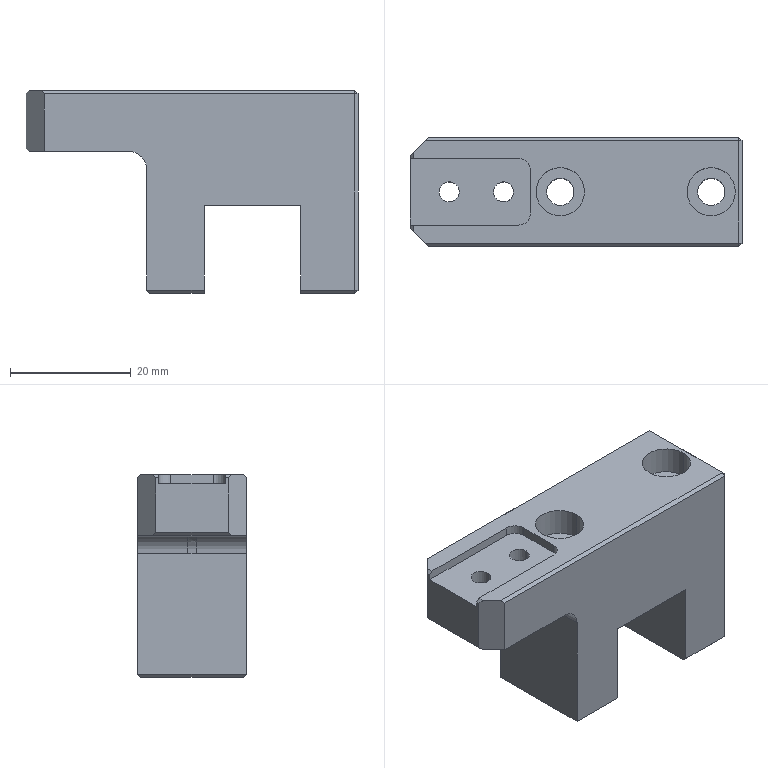Component | SolidWorks | LowerRollerFixedSeat-1 | 1 solid | 55 faces | volume 18585 mm3 | plane 38 | cylinder 16 | spline 1 | commonest cylinder face diameters 3.3 x4 4.5 x4 8 x4 6 x2 4 x2